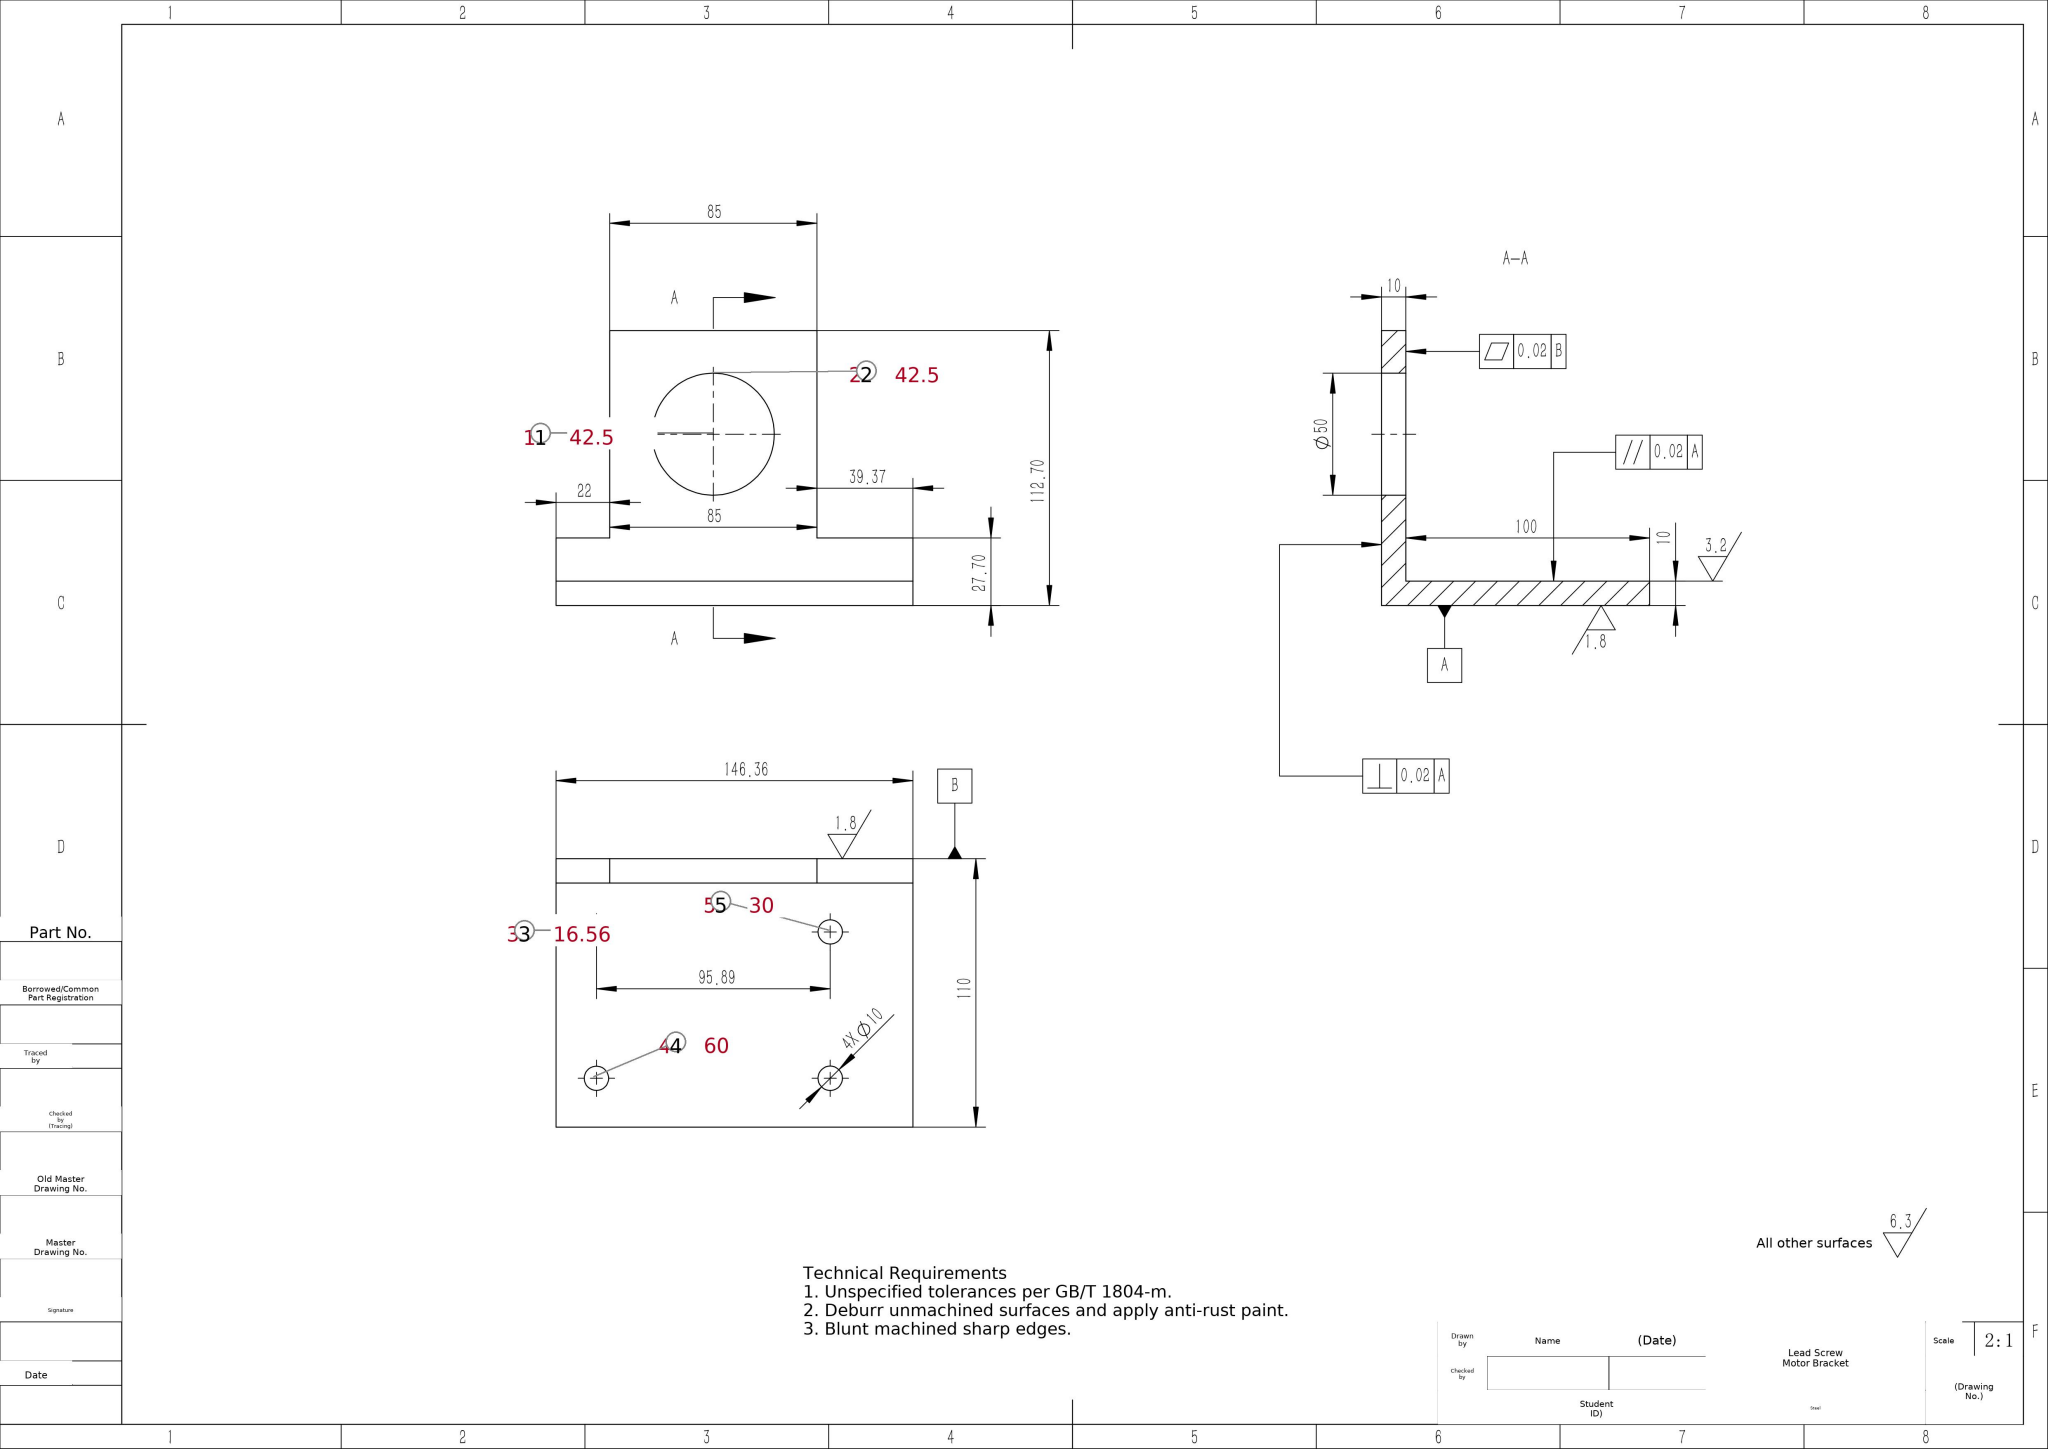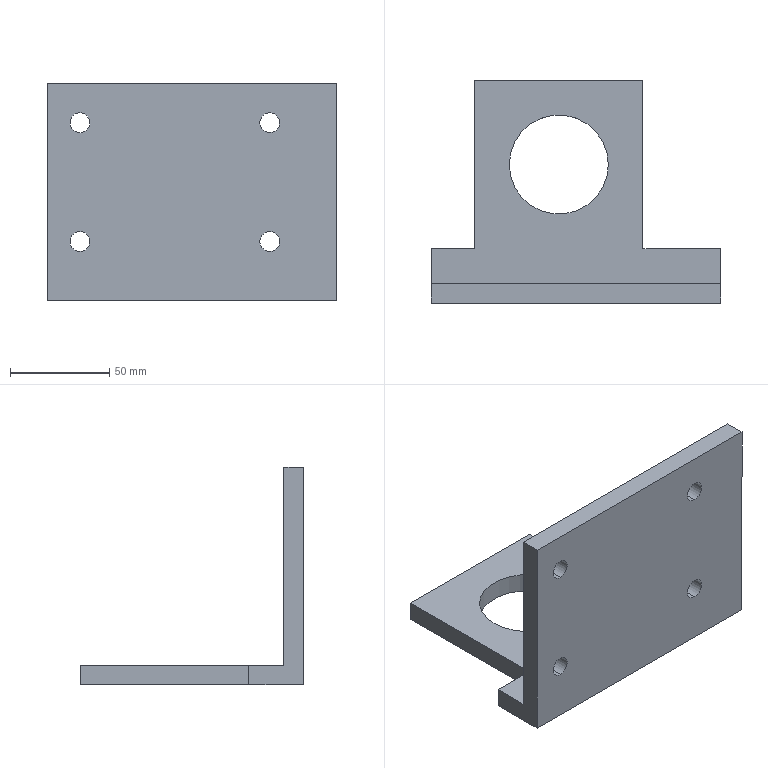Part | SolidWorks | mm | material Steel | 1 solid | 22 faces | box 146.36 x 112.7 x 110 mm | volume 236379 mm3 | plane 12 | cylinder 10 | commonest cylinder face diameters 10 x8 50 x2
STEP:
#1=CARTESIAN_POINT('',(-47.944,-70.2,85.));
#2=VERTEX_POINT('',#1);
#3=CARTESIAN_POINT('',(-47.944,-70.2,95.));
#4=VERTEX_POINT('',#3);
#5=CARTESIAN_POINT('',(-47.944,-70.2,90.));
#6=DIRECTION('',(0.,1.,0.));
#7=DIRECTION('',(0.,0.,1.));
#8=AXIS2_PLACEMENT_3D('',#5,#6,#7);
#9=CIRCLE('',#8,5.);
#10=EDGE_CURVE('',#2,#4,#9,.T.);
#11=ORIENTED_EDGE('',*,*,#10,.F.);
#12=CARTESIAN_POINT('',(-47.944,-60.2,85.));
#13=VERTEX_POINT('',#12);
#14=CARTESIAN_POINT('',(-47.944,-70.2,85.));
#15=DIRECTION('',(0.,1.,0.));
#16=VECTOR('',#15,1000.);
#17=LINE('',#14,#16);
#18=EDGE_CURVE('',#2,#13,#17,.T.);
#19=ORIENTED_EDGE('',*,*,#18,.T.);
#20=CARTESIAN_POINT('',(-47.944,-60.2,95.));
#21=VERTEX_POINT('',#20);
#22=CARTESIAN_POINT('',(-47.944,-60.2,90.));
#23=DIRECTION('',(0.,1.,0.));
#24=DIRECTION('',(0.,0.,1.));
#25=AXIS2_PLACEMENT_3D('',#22,#23,#24);
#26=CIRCLE('',#25,5.);
#27=EDGE_CURVE('',#13,#21,#26,.T.);
#28=ORIENTED_EDGE('',*,*,#27,.T.);
#29=CARTESIAN_POINT('',(-47.944,-70.2,95.));
#30=DIRECTION('',(0.,1.,0.));
#31=VECTOR('',#30,1000.);
#32=LINE('',#29,#31);
#33=EDGE_CURVE('',#4,#21,#32,.T.);
#34=ORIENTED_EDGE('',*,*,#33,.F.);
#35=EDGE_LOOP('',(#11,#19,#28,#34));
#36=FACE_OUTER_BOUND('',#35,.T.);
#37=CARTESIAN_POINT('',(-47.944,-70.2,90.));
#38=DIRECTION('',(0.,1.,0.));
#39=DIRECTION('',(0.,0.,1.));
#40=AXIS2_PLACEMENT_3D('',#37,#38,#39);
#41=CYLINDRICAL_SURFACE('',#40,5.);
#42=ADVANCED_FACE('',(#36),#41,.F.);
#43=CARTESIAN_POINT('',(47.944,-70.2,85.));
#44=VERTEX_POINT('',#43);
#45=CARTESIAN_POINT('',(47.944,-70.2,95.));
#46=VERTEX_POINT('',#45);
#47=CARTESIAN_POINT('',(47.944,-70.2,90.));
#48=DIRECTION('',(0.,1.,0.));
#49=DIRECTION('',(0.,0.,-1.));
#50=AXIS2_PLACEMENT_3D('',#47,#48,#49);
#51=CIRCLE('',#50,5.);
#52=EDGE_CURVE('',#44,#46,#51,.T.);
#53=ORIENTED_EDGE('',*,*,#52,.F.);
#54=CARTESIAN_POINT('',(47.944,-60.2,85.));
#55=VERTEX_POINT('',#54);
#56=CARTESIAN_POINT('',(47.944,-70.2,85.));
#57=DIRECTION('',(0.,1.,0.));
#58=VECTOR('',#57,1000.);
#59=LINE('',#56,#58);
#60=EDGE_CURVE('',#44,#55,#59,.T.);
#61=ORIENTED_EDGE('',*,*,#60,.T.);
#62=CARTESIAN_POINT('',(47.944,-60.2,95.));
#63=VERTEX_POINT('',#62);
#64=CARTESIAN_POINT('',(47.944,-60.2,90.));
#65=DIRECTION('',(0.,1.,0.));
#66=DIRECTION('',(0.,0.,-1.));
#67=AXIS2_PLACEMENT_3D('',#64,#65,#66);
#68=CIRCLE('',#67,5.);
#69=EDGE_CURVE('',#55,#63,#68,.T.);
#70=ORIENTED_EDGE('',*,*,#69,.T.);
#71=CARTESIAN_POINT('',(47.944,-70.2,95.));
#72=DIRECTION('',(0.,1.,0.));
#73=VECTOR('',#72,1000.);
#74=LINE('',#71,#73);
#75=EDGE_CURVE('',#46,#63,#74,.T.);
#76=ORIENTED_EDGE('',*,*,#75,.F.);
#77=EDGE_LOOP('',(#53,#61,#70,#76));
#78=FACE_OUTER_BOUND('',#77,.T.);
#79=CARTESIAN_POINT('',(47.944,-70.2,90.));
#80=DIRECTION('',(0.,1.,0.));
#81=DIRECTION('',(0.,0.,1.));
#82=AXIS2_PLACEMENT_3D('',#79,#80,#81);
#83=CYLINDRICAL_SURFACE('',#82,5.);
#84=ADVANCED_FACE('',(#78),#83,.F.);
#85=CARTESIAN_POINT('',(47.944,-70.2,25.));
#86=VERTEX_POINT('',#85);
#87=CARTESIAN_POINT('',(47.944,-70.2,35.));
#88=VERTEX_POINT('',#87);
#89=CARTESIAN_POINT('',(47.944,-70.2,30.));
#90=DIRECTION('',(0.,1.,0.));
#91=DIRECTION('',(0.,0.,-1.));
#92=AXIS2_PLACEMENT_3D('',#89,#90,#91);
#93=CIRCLE('',#92,5.);
#94=EDGE_CURVE('',#86,#88,#93,.T.);
#95=ORIENTED_EDGE('',*,*,#94,.F.);
#96=CARTESIAN_POINT('',(47.944,-60.2,25.));
#97=VERTEX_POINT('',#96);
#98=CARTESIAN_POINT('',(47.944,-70.2,25.));
#99=DIRECTION('',(0.,1.,0.));
#100=VECTOR('',#99,1000.);
#101=LINE('',#98,#100);
#102=EDGE_CURVE('',#86,#97,#101,.T.);
#103=ORIENTED_EDGE('',*,*,#102,.T.);
#104=CARTESIAN_POINT('',(47.944,-60.2,35.));
#105=VERTEX_POINT('',#104);
#106=CARTESIAN_POINT('',(47.944,-60.2,30.));
#107=DIRECTION('',(0.,1.,0.));
#108=DIRECTION('',(0.,0.,-1.));
#109=AXIS2_PLACEMENT_3D('',#106,#107,#108);
#110=CIRCLE('',#109,5.);
#111=EDGE_CURVE('',#97,#105,#110,.T.);
#112=ORIENTED_EDGE('',*,*,#111,.T.);
#113=CARTESIAN_POINT('',(47.944,-70.2,35.));
#114=DIRECTION('',(0.,1.,0.));
#115=VECTOR('',#114,1000.);
#116=LINE('',#113,#115);
#117=EDGE_CURVE('',#88,#105,#116,.T.);
#118=ORIENTED_EDGE('',*,*,#117,.F.);
#119=EDGE_LOOP('',(#95,#103,#112,#118));
#120=FACE_OUTER_BOUND('',#119,.T.);
#121=CARTESIAN_POINT('',(47.944,-70.2,30.));
#122=DIRECTION('',(0.,1.,0.));
#123=DIRECTION('',(0.,0.,1.));
#124=AXIS2_PLACEMENT_3D('',#121,#122,#123);
#125=CYLINDRICAL_SURFACE('',#124,5.);
#126=ADVANCED_FACE('',(#120),#125,.F.);
#127=CARTESIAN_POINT('',(-47.944,-70.2,25.));
#128=VERTEX_POINT('',#127);
#129=CARTESIAN_POINT('',(-47.944,-70.2,35.));
#130=VERTEX_POINT('',#129);
#131=CARTESIAN_POINT('',(-47.944,-70.2,30.));
#132=DIRECTION('',(0.,1.,0.));
#133=DIRECTION('',(0.,0.,1.));
#134=AXIS2_PLACEMENT_3D('',#131,#132,#133);
#135=CIRCLE('',#134,5.);
#136=EDGE_CURVE('',#128,#130,#135,.T.);
#137=ORIENTED_EDGE('',*,*,#136,.F.);
#138=CARTESIAN_POINT('',(-47.944,-60.2,25.));
#139=VERTEX_POINT('',#138);
#140=CARTESIAN_POINT('',(-47.944,-70.2,25.));
#141=DIRECTION('',(0.,1.,0.));
#142=VECTOR('',#141,1000.);
#143=LINE('',#140,#142);
#144=EDGE_CURVE('',#128,#139,#143,.T.);
#145=ORIENTED_EDGE('',*,*,#144,.T.);
#146=CARTESIAN_POINT('',(-47.944,-60.2,35.));
#147=VERTEX_POINT('',#146);
#148=CARTESIAN_POINT('',(-47.944,-60.2,30.));
#149=DIRECTION('',(0.,1.,0.));
#150=DIRECTION('',(0.,0.,1.));
#151=AXIS2_PLACEMENT_3D('',#148,#149,#150);
#152=CIRCLE('',#151,5.);
#153=EDGE_CURVE('',#139,#147,#152,.T.);
#154=ORIENTED_EDGE('',*,*,#153,.T.);
#155=CARTESIAN_POINT('',(-47.944,-70.2,35.));
#156=DIRECTION('',(0.,1.,0.));
#157=VECTOR('',#156,1000.);
#158=LINE('',#155,#157);
#159=EDGE_CURVE('',#130,#147,#158,.T.);
#160=ORIENTED_EDGE('',*,*,#159,.F.);
#161=EDGE_LOOP('',(#137,#145,#154,#160));
#162=FACE_OUTER_BOUND('',#161,.T.);
#163=CARTESIAN_POINT('',(-47.944,-70.2,30.));
#164=DIRECTION('',(0.,1.,0.));
#165=DIRECTION('',(0.,0.,1.));
#166=AXIS2_PLACEMENT_3D('',#163,#164,#165);
#167=CYLINDRICAL_SURFACE('',#166,5.);
#168=ADVANCED_FACE('',(#162),#167,.F.);
#169=CARTESIAN_POINT('',(-25.,0.,10.));
#170=VERTEX_POINT('',#169);
#171=CARTESIAN_POINT('',(25.,0.,10.));
#172=VERTEX_POINT('',#171);
#173=CARTESIAN_POINT('',(0.,0.,10.));
#174=DIRECTION('',(0.,0.,1.));
#175=DIRECTION('',(1.,0.,0.));
#176=AXIS2_PLACEMENT_3D('',#173,#174,#175);
#177=CIRCLE('',#176,25.);
#178=EDGE_CURVE('',#170,#172,#177,.T.);
#179=ORIENTED_EDGE('',*,*,#178,.T.);
#180=CARTESIAN_POINT('',(25.,0.,0.));
#181=VERTEX_POINT('',#180);
#182=CARTESIAN_POINT('',(25.,0.,10.));
#183=DIRECTION('',(0.,0.,-1.));
#184=VECTOR('',#183,1000.);
#185=LINE('',#182,#184);
#186=EDGE_CURVE('',#172,#181,#185,.T.);
#187=ORIENTED_EDGE('',*,*,#186,.T.);
#188=CARTESIAN_POINT('',(-25.,0.,0.));
#189=VERTEX_POINT('',#188);
#190=CARTESIAN_POINT('',(0.,0.,0.));
#191=DIRECTION('',(0.,0.,1.));
#192=DIRECTION('',(1.,0.,0.));
#193=AXIS2_PLACEMENT_3D('',#190,#191,#192);
#194=CIRCLE('',#193,25.);
#195=EDGE_CURVE('',#189,#181,#194,.T.);
#196=ORIENTED_EDGE('',*,*,#195,.F.);
#197=CARTESIAN_POINT('',(-25.,0.,10.));
#198=DIRECTION('',(0.,0.,-1.));
#199=VECTOR('',#198,1000.);
#200=LINE('',#197,#199);
#201=EDGE_CURVE('',#170,#189,#200,.T.);
#202=ORIENTED_EDGE('',*,*,#201,.F.);
#203=EDGE_LOOP('',(#179,#187,#196,#202));
#204=FACE_OUTER_BOUND('',#203,.T.);
#205=CARTESIAN_POINT('',(0.,0.,10.));
#206=DIRECTION('',(0.,0.,-1.));
#207=DIRECTION('',(-1.,0.,0.));
#208=AXIS2_PLACEMENT_3D('',#205,#206,#207);
#209=CYLINDRICAL_SURFACE('',#208,25.);
#210=ADVANCED_FACE('',(#204),#209,.F.);
#211=ORIENTED_EDGE('',*,*,#178,.F.);
#212=CARTESIAN_POINT('',(0.,0.,10.));
#213=DIRECTION('',(0.,0.,1.));
#214=DIRECTION('',(1.,0.,0.));
#215=AXIS2_PLACEMENT_3D('',#212,#213,#214);
#216=CIRCLE('',#215,25.);
#217=EDGE_CURVE('',#172,#170,#216,.T.);
#218=ORIENTED_EDGE('',*,*,#217,.F.);
#219=EDGE_LOOP('',(#211,#218));
#220=FACE_BOUND('',#219,.T.);
#221=CARTESIAN_POINT('',(-42.5,-42.5,10.));
#222=VERTEX_POINT('',#221);
#223=CARTESIAN_POINT('',(-64.496,-42.5,10.));
#224=VERTEX_POINT('',#223);
#225=CARTESIAN_POINT('',(-42.5,-42.5,10.));
#226=DIRECTION('',(-1.,0.,0.));
#227=VECTOR('',#226,1000.);
#228=LINE('',#225,#227);
#229=EDGE_CURVE('',#222,#224,#228,.T.);
#230=ORIENTED_EDGE('',*,*,#229,.T.);
#231=CARTESIAN_POINT('',(-64.496,-60.2,10.));
#232=VERTEX_POINT('',#231);
#233=CARTESIAN_POINT('',(-64.496,-60.2,10.));
#234=DIRECTION('',(0.,1.,0.));
#235=VECTOR('',#234,1000.);
#236=LINE('',#233,#235);
#237=EDGE_CURVE('',#232,#224,#236,.T.);
#238=ORIENTED_EDGE('',*,*,#237,.F.);
#239=CARTESIAN_POINT('',(81.866,-60.2,10.));
#240=VERTEX_POINT('',#239);
#241=CARTESIAN_POINT('',(-81.866,-60.2,10.));
#242=DIRECTION('',(-1.,0.,0.));
#243=VECTOR('',#242,1000.);
#244=LINE('',#241,#243);
#245=EDGE_CURVE('',#240,#232,#244,.T.);
#246=ORIENTED_EDGE('',*,*,#245,.F.);
#247=CARTESIAN_POINT('',(81.866,-42.5,10.));
#248=VERTEX_POINT('',#247);
#249=CARTESIAN_POINT('',(81.866,-42.5,10.));
#250=DIRECTION('',(-0.,1.,0.));
#251=VECTOR('',#250,1000.);
#252=LINE('',#249,#251);
#253=EDGE_CURVE('',#240,#248,#252,.T.);
#254=ORIENTED_EDGE('',*,*,#253,.T.);
#255=CARTESIAN_POINT('',(42.5,-42.5,10.));
#256=VERTEX_POINT('',#255);
#257=CARTESIAN_POINT('',(42.5,-42.5,10.));
#258=DIRECTION('',(-1.,-0.,0.));
#259=VECTOR('',#258,1000.);
#260=LINE('',#257,#259);
#261=EDGE_CURVE('',#248,#256,#260,.T.);
#262=ORIENTED_EDGE('',*,*,#261,.T.);
#263=CARTESIAN_POINT('',(42.5,42.5,10.));
#264=VERTEX_POINT('',#263);
#265=CARTESIAN_POINT('',(42.5,42.5,10.));
#266=DIRECTION('',(-0.,1.,0.));
#267=VECTOR('',#266,1000.);
#268=LINE('',#265,#267);
#269=EDGE_CURVE('',#256,#264,#268,.T.);
#270=ORIENTED_EDGE('',*,*,#269,.T.);
#271=CARTESIAN_POINT('',(-42.5,42.5,10.));
#272=VERTEX_POINT('',#271);
#273=CARTESIAN_POINT('',(42.5,42.5,10.));
#274=DIRECTION('',(-1.,-0.,0.));
#275=VECTOR('',#274,1000.);
#276=LINE('',#273,#275);
#277=EDGE_CURVE('',#264,#272,#276,.T.);
#278=ORIENTED_EDGE('',*,*,#277,.T.);
#279=CARTESIAN_POINT('',(-42.5,42.5,10.));
#280=DIRECTION('',(0.,-1.,0.));
#281=VECTOR('',#280,1000.);
#282=LINE('',#279,#281);
#283=EDGE_CURVE('',#272,#222,#282,.T.);
#284=ORIENTED_EDGE('',*,*,#283,.T.);
#285=EDGE_LOOP('',(#230,#238,#246,#254,#262,#270,#278,#284));
#286=FACE_OUTER_BOUND('',#285,.T.);
#287=CARTESIAN_POINT('',(0.,0.,10.));
#288=DIRECTION('',(0.,0.,1.));
#289=DIRECTION('',(1.,0.,0.));
#290=AXIS2_PLACEMENT_3D('',#287,#288,#289);
#291=PLANE('',#290);
#292=ADVANCED_FACE('',(#220,#286),#291,.T.);
#293=ORIENTED_EDGE('',*,*,#195,.T.);
#294=CARTESIAN_POINT('',(0.,0.,0.));
#295=DIRECTION('',(0.,0.,1.));
#296=DIRECTION('',(1.,0.,0.));
#297=AXIS2_PLACEMENT_3D('',#294,#295,#296);
#298=CIRCLE('',#297,25.);
#299=EDGE_CURVE('',#181,#189,#298,.T.);
#300=ORIENTED_EDGE('',*,*,#299,.T.);
#301=EDGE_LOOP('',(#293,#300));
#302=FACE_BOUND('',#301,.T.);
#303=CARTESIAN_POINT('',(-64.496,-42.5,0.));
#304=VERTEX_POINT('',#303);
#305=CARTESIAN_POINT('',(-64.496,-70.2,0.));
#306=VERTEX_POINT('',#305);
#307=CARTESIAN_POINT('',(-64.496,-42.5,0.));
#308=DIRECTION('',(0.,-1.,0.));
#309=VECTOR('',#308,1000.);
#310=LINE('',#307,#309);
#311=EDGE_CURVE('',#304,#306,#310,.T.);
#312=ORIENTED_EDGE('',*,*,#311,.F.);
#313=CARTESIAN_POINT('',(-42.5,-42.5,0.));
#314=VERTEX_POINT('',#313);
#315=CARTESIAN_POINT('',(-42.5,-42.5,0.));
#316=DIRECTION('',(-1.,0.,0.));
#317=VECTOR('',#316,1000.);
#318=LINE('',#315,#317);
#319=EDGE_CURVE('',#314,#304,#318,.T.);
#320=ORIENTED_EDGE('',*,*,#319,.F.);
#321=CARTESIAN_POINT('',(-42.5,42.5,0.));
#322=VERTEX_POINT('',#321);
#323=CARTESIAN_POINT('',(-42.5,42.5,0.));
#324=DIRECTION('',(0.,-1.,0.));
#325=VECTOR('',#324,1000.);
#326=LINE('',#323,#325);
#327=EDGE_CURVE('',#322,#314,#326,.T.);
#328=ORIENTED_EDGE('',*,*,#327,.F.);
#329=CARTESIAN_POINT('',(42.5,42.5,0.));
#330=VERTEX_POINT('',#329);
#331=CARTESIAN_POINT('',(42.5,42.5,0.));
#332=DIRECTION('',(-1.,-0.,0.));
#333=VECTOR('',#332,1000.);
#334=LINE('',#331,#333);
#335=EDGE_CURVE('',#330,#322,#334,.T.);
#336=ORIENTED_EDGE('',*,*,#335,.F.);
#337=CARTESIAN_POINT('',(42.5,-42.5,0.));
#338=VERTEX_POINT('',#337);
#339=CARTESIAN_POINT('',(42.5,42.5,0.));
#340=DIRECTION('',(-0.,1.,0.));
#341=VECTOR('',#340,1000.);
#342=LINE('',#339,#341);
#343=EDGE_CURVE('',#338,#330,#342,.T.);
#344=ORIENTED_EDGE('',*,*,#343,.F.);
#345=CARTESIAN_POINT('',(81.866,-42.5,0.));
#346=VERTEX_POINT('',#345);
#347=CARTESIAN_POINT('',(42.5,-42.5,0.));
#348=DIRECTION('',(-1.,-0.,0.));
#349=VECTOR('',#348,1000.);
#350=LINE('',#347,#349);
#351=EDGE_CURVE('',#346,#338,#350,.T.);
#352=ORIENTED_EDGE('',*,*,#351,.F.);
#353=CARTESIAN_POINT('',(81.866,-70.2,0.));
#354=VERTEX_POINT('',#353);
#355=CARTESIAN_POINT('',(81.866,-42.5,0.));
#356=DIRECTION('',(-0.,1.,0.));
#357=VECTOR('',#356,1000.);
#358=LINE('',#355,#357);
#359=EDGE_CURVE('',#354,#346,#358,.T.);
#360=ORIENTED_EDGE('',*,*,#359,.F.);
#361=CARTESIAN_POINT('',(-81.866,-70.2,0.));
#362=DIRECTION('',(1.,0.,0.));
#363=VECTOR('',#362,1000.);
#364=LINE('',#361,#363);
#365=EDGE_CURVE('',#306,#354,#364,.T.);
#366=ORIENTED_EDGE('',*,*,#365,.F.);
#367=EDGE_LOOP('',(#312,#320,#328,#336,#344,#352,#360,#366));
#368=FACE_OUTER_BOUND('',#367,.T.);
#369=CARTESIAN_POINT('',(0.,0.,0.));
#370=DIRECTION('',(0.,0.,1.));
#371=DIRECTION('',(1.,0.,0.));
#372=AXIS2_PLACEMENT_3D('',#369,#370,#371);
#373=PLANE('',#372);
#374=ADVANCED_FACE('',(#302,#368),#373,.F.);
#375=CARTESIAN_POINT('',(-64.496,-42.5,10.));
#376=DIRECTION('',(0.,0.,-1.));
#377=VECTOR('',#376,1000.);
#378=LINE('',#375,#377);
#379=EDGE_CURVE('',#224,#304,#378,.T.);
#380=ORIENTED_EDGE('',*,*,#379,.F.);
#381=ORIENTED_EDGE('',*,*,#229,.F.);
#382=CARTESIAN_POINT('',(-42.5,-42.5,10.));
#383=DIRECTION('',(0.,0.,-1.));
#384=VECTOR('',#383,1000.);
#385=LINE('',#382,#384);
#386=EDGE_CURVE('',#222,#314,#385,.T.);
#387=ORIENTED_EDGE('',*,*,#386,.T.);
#388=ORIENTED_EDGE('',*,*,#319,.T.);
#389=EDGE_LOOP('',(#380,#381,#387,#388));
#390=FACE_OUTER_BOUND('',#389,.T.);
#391=CARTESIAN_POINT('',(-42.5,-42.5,10.));
#392=DIRECTION('',(0.,-1.,0.));
#393=DIRECTION('',(0.,0.,-1.));
#394=AXIS2_PLACEMENT_3D('',#391,#392,#393);
#395=PLANE('',#394);
#396=ADVANCED_FACE('',(#390),#395,.F.);
#397=CARTESIAN_POINT('',(-47.944,-70.2,90.));
#398=DIRECTION('',(0.,1.,0.));
#399=DIRECTION('',(0.,0.,1.));
#400=AXIS2_PLACEMENT_3D('',#397,#398,#399);
#401=CIRCLE('',#400,5.);
#402=EDGE_CURVE('',#4,#2,#401,.T.);
#403=ORIENTED_EDGE('',*,*,#402,.T.);
#404=ORIENTED_EDGE('',*,*,#10,.T.);
#405=EDGE_LOOP('',(#403,#404));
#406=FACE_BOUND('',#405,.T.);
#407=CARTESIAN_POINT('',(47.944,-70.2,90.));
#408=DIRECTION('',(0.,1.,0.));
#409=DIRECTION('',(0.,0.,-1.));
#410=AXIS2_PLACEMENT_3D('',#407,#408,#409);
#411=CIRCLE('',#410,5.);
#412=EDGE_CURVE('',#46,#44,#411,.T.);
#413=ORIENTED_EDGE('',*,*,#412,.T.);
#414=ORIENTED_EDGE('',*,*,#52,.T.);
#415=EDGE_LOOP('',(#413,#414));
#416=FACE_BOUND('',#415,.T.);
#417=CARTESIAN_POINT('',(47.944,-70.2,30.));
#418=DIRECTION('',(0.,1.,0.));
#419=DIRECTION('',(0.,0.,-1.));
#420=AXIS2_PLACEMENT_3D('',#417,#418,#419);
#421=CIRCLE('',#420,5.);
#422=EDGE_CURVE('',#88,#86,#421,.T.);
#423=ORIENTED_EDGE('',*,*,#422,.T.);
#424=ORIENTED_EDGE('',*,*,#94,.T.);
#425=EDGE_LOOP('',(#423,#424));
#426=FACE_BOUND('',#425,.T.);
#427=CARTESIAN_POINT('',(-47.944,-70.2,30.));
#428=DIRECTION('',(0.,1.,0.));
#429=DIRECTION('',(0.,0.,1.));
#430=AXIS2_PLACEMENT_3D('',#427,#428,#429);
#431=CIRCLE('',#430,5.);
#432=EDGE_CURVE('',#130,#128,#431,.T.);
#433=ORIENTED_EDGE('',*,*,#432,.T.);
#434=ORIENTED_EDGE('',*,*,#136,.T.);
#435=EDGE_LOOP('',(#433,#434));
#436=FACE_BOUND('',#435,.T.);
#437=CARTESIAN_POINT('',(-64.496,-70.2,110.));
#438=VERTEX_POINT('',#437);
#439=CARTESIAN_POINT('',(-64.496,-70.2,0.));
#440=DIRECTION('',(0.,0.,1.));
#441=VECTOR('',#440,1000.);
#442=LINE('',#439,#441);
#443=EDGE_CURVE('',#306,#438,#442,.T.);
#444=ORIENTED_EDGE('',*,*,#443,.F.);
#445=ORIENTED_EDGE('',*,*,#365,.T.);
#446=CARTESIAN_POINT('',(81.866,-70.2,110.));
#447=VERTEX_POINT('',#446);
#448=CARTESIAN_POINT('',(81.866,-70.2,10.));
#449=DIRECTION('',(0.,0.,-1.));
#450=VECTOR('',#449,1000.);
#451=LINE('',#448,#450);
#452=EDGE_CURVE('',#447,#354,#451,.T.);
#453=ORIENTED_EDGE('',*,*,#452,.F.);
#454=CARTESIAN_POINT('',(-81.866,-70.2,110.));
#455=DIRECTION('',(1.,0.,0.));
#456=VECTOR('',#455,1000.);
#457=LINE('',#454,#456);
#458=EDGE_CURVE('',#438,#447,#457,.T.);
#459=ORIENTED_EDGE('',*,*,#458,.F.);
#460=EDGE_LOOP('',(#444,#445,#453,#459));
#461=FACE_OUTER_BOUND('',#460,.T.);
#462=CARTESIAN_POINT('',(-81.866,-70.2,10.));
#463=DIRECTION('',(-0.,1.,0.));
#464=DIRECTION('',(-1.,-0.,0.));
#465=AXIS2_PLACEMENT_3D('',#462,#463,#464);
#466=PLANE('',#465);
#467=ADVANCED_FACE('',(#406,#416,#426,#436,#461),#466,.F.);
#468=CARTESIAN_POINT('',(-47.944,-60.2,90.));
#469=DIRECTION('',(0.,1.,0.));
#470=DIRECTION('',(0.,0.,1.));
#471=AXIS2_PLACEMENT_3D('',#468,#469,#470);
#472=CIRCLE('',#471,5.);
#473=EDGE_CURVE('',#21,#13,#472,.T.);
#474=ORIENTED_EDGE('',*,*,#473,.F.);
#475=ORIENTED_EDGE('',*,*,#27,.F.);
#476=EDGE_LOOP('',(#474,#475));
#477=FACE_BOUND('',#476,.T.);
#478=CARTESIAN_POINT('',(47.944,-60.2,90.));
#479=DIRECTION('',(0.,1.,0.));
#480=DIRECTION('',(0.,0.,-1.));
#481=AXIS2_PLACEMENT_3D('',#478,#479,#480);
#482=CIRCLE('',#481,5.);
#483=EDGE_CURVE('',#63,#55,#482,.T.);
#484=ORIENTED_EDGE('',*,*,#483,.F.);
#485=ORIENTED_EDGE('',*,*,#69,.F.);
#486=EDGE_LOOP('',(#484,#485));
#487=FACE_BOUND('',#486,.T.);
#488=CARTESIAN_POINT('',(47.944,-60.2,30.));
#489=DIRECTION('',(0.,1.,0.));
#490=DIRECTION('',(0.,0.,-1.));
#491=AXIS2_PLACEMENT_3D('',#488,#489,#490);
#492=CIRCLE('',#491,5.);
#493=EDGE_CURVE('',#105,#97,#492,.T.);
#494=ORIENTED_EDGE('',*,*,#493,.F.);
#495=ORIENTED_EDGE('',*,*,#111,.F.);
#496=EDGE_LOOP('',(#494,#495));
#497=FACE_BOUND('',#496,.T.);
#498=CARTESIAN_POINT('',(-47.944,-60.2,30.));
#499=DIRECTION('',(0.,1.,0.));
#500=DIRECTION('',(0.,0.,1.));
#501=AXIS2_PLACEMENT_3D('',#498,#499,#500);
#502=CIRCLE('',#501,5.);
#503=EDGE_CURVE('',#147,#139,#502,.T.);
#504=ORIENTED_EDGE('',*,*,#503,.F.);
#505=ORIENTED_EDGE('',*,*,#153,.F.);
#506=EDGE_LOOP('',(#504,#505));
#507=FACE_BOUND('',#506,.T.);
#508=CARTESIAN_POINT('',(-64.496,-60.2,110.));
#509=VERTEX_POINT('',#508);
#510=CARTESIAN_POINT('',(-64.496,-60.2,110.));
#511=DIRECTION('',(0.,0.,-1.));
#512=VECTOR('',#511,1000.);
#513=LINE('',#510,#512);
#514=EDGE_CURVE('',#509,#232,#513,.T.);
#515=ORIENTED_EDGE('',*,*,#514,.F.);
#516=CARTESIAN_POINT('',(81.866,-60.2,110.));
#517=VERTEX_POINT('',#516);
#518=CARTESIAN_POINT('',(-81.866,-60.2,110.));
#519=DIRECTION('',(-1.,0.,0.));
#520=VECTOR('',#519,1000.);
#521=LINE('',#518,#520);
#522=EDGE_CURVE('',#517,#509,#521,.T.);
#523=ORIENTED_EDGE('',*,*,#522,.F.);
#524=CARTESIAN_POINT('',(81.866,-60.2,110.));
#525=DIRECTION('',(0.,0.,-1.));
#526=VECTOR('',#525,1000.);
#527=LINE('',#524,#526);
#528=EDGE_CURVE('',#517,#240,#527,.T.);
#529=ORIENTED_EDGE('',*,*,#528,.T.);
#530=ORIENTED_EDGE('',*,*,#245,.T.);
#531=EDGE_LOOP('',(#515,#523,#529,#530));
#532=FACE_OUTER_BOUND('',#531,.T.);
#533=CARTESIAN_POINT('',(-81.866,-60.2,110.));
#534=DIRECTION('',(0.,-1.,0.));
#535=DIRECTION('',(0.,0.,-1.));
#536=AXIS2_PLACEMENT_3D('',#533,#534,#535);
#537=PLANE('',#536);
#538=ADVANCED_FACE('',(#477,#487,#497,#507,#532),#537,.F.);
#539=CARTESIAN_POINT('',(-64.496,-70.2,110.));
#540=DIRECTION('',(0.,1.,0.));
#541=VECTOR('',#540,1000.);
#542=LINE('',#539,#541);
#543=EDGE_CURVE('',#438,#509,#542,.T.);
#544=ORIENTED_EDGE('',*,*,#543,.F.);
#545=ORIENTED_EDGE('',*,*,#458,.T.);
#546=CARTESIAN_POINT('',(81.866,-70.2,110.));
#547=DIRECTION('',(0.,1.,0.));
#548=VECTOR('',#547,1000.);
#549=LINE('',#546,#548);
#550=EDGE_CURVE('',#447,#517,#549,.T.);
#551=ORIENTED_EDGE('',*,*,#550,.T.);
#552=ORIENTED_EDGE('',*,*,#522,.T.);
#553=EDGE_LOOP('',(#544,#545,#551,#552));
#554=FACE_OUTER_BOUND('',#553,.T.);
#555=CARTESIAN_POINT('',(0.,0.,110.));
#556=DIRECTION('',(0.,0.,-1.));
#557=DIRECTION('',(-1.,0.,0.));
#558=AXIS2_PLACEMENT_3D('',#555,#556,#557);
#559=PLANE('',#558);
#560=ADVANCED_FACE('',(#554),#559,.F.);
#561=ORIENTED_EDGE('',*,*,#359,.T.);
#562=CARTESIAN_POINT('',(81.866,-42.5,10.));
#563=DIRECTION('',(0.,0.,-1.));
#564=VECTOR('',#563,1000.);
#565=LINE('',#562,#564);
#566=EDGE_CURVE('',#248,#346,#565,.T.);
#567=ORIENTED_EDGE('',*,*,#566,.F.);
#568=ORIENTED_EDGE('',*,*,#253,.F.);
#569=ORIENTED_EDGE('',*,*,#528,.F.);
#570=ORIENTED_EDGE('',*,*,#550,.F.);
#571=ORIENTED_EDGE('',*,*,#452,.T.);
#572=EDGE_LOOP('',(#561,#567,#568,#569,#570,#571));
#573=FACE_OUTER_BOUND('',#572,.T.);
#574=CARTESIAN_POINT('',(81.866,-42.5,10.));
#575=DIRECTION('',(-1.,-0.,0.));
#576=DIRECTION('',(0.,-1.,0.));
#577=AXIS2_PLACEMENT_3D('',#574,#575,#576);
#578=PLANE('',#577);
#579=ADVANCED_FACE('',(#573),#578,.F.);
#580=ORIENTED_EDGE('',*,*,#351,.T.);
#581=CARTESIAN_POINT('',(42.5,-42.5,10.));
#582=DIRECTION('',(0.,0.,-1.));
#583=VECTOR('',#582,1000.);
#584=LINE('',#581,#583);
#585=EDGE_CURVE('',#256,#338,#584,.T.);
#586=ORIENTED_EDGE('',*,*,#585,.F.);
#587=ORIENTED_EDGE('',*,*,#261,.F.);
#588=ORIENTED_EDGE('',*,*,#566,.T.);
#589=EDGE_LOOP('',(#580,#586,#587,#588));
#590=FACE_OUTER_BOUND('',#589,.T.);
#591=CARTESIAN_POINT('',(42.5,-42.5,10.));
#592=DIRECTION('',(0.,-1.,0.));
#593=DIRECTION('',(1.,0.,0.));
#594=AXIS2_PLACEMENT_3D('',#591,#592,#593);
#595=PLANE('',#594);
#596=ADVANCED_FACE('',(#590),#595,.F.);
#597=ORIENTED_EDGE('',*,*,#343,.T.);
#598=CARTESIAN_POINT('',(42.5,42.5,10.));
#599=DIRECTION('',(0.,0.,-1.));
#600=VECTOR('',#599,1000.);
#601=LINE('',#598,#600);
#602=EDGE_CURVE('',#264,#330,#601,.T.);
#603=ORIENTED_EDGE('',*,*,#602,.F.);
#604=ORIENTED_EDGE('',*,*,#269,.F.);
#605=ORIENTED_EDGE('',*,*,#585,.T.);
#606=EDGE_LOOP('',(#597,#603,#604,#605));
#607=FACE_OUTER_BOUND('',#606,.T.);
#608=CARTESIAN_POINT('',(42.5,42.5,10.));
#609=DIRECTION('',(-1.,-0.,0.));
#610=DIRECTION('',(0.,-1.,0.));
#611=AXIS2_PLACEMENT_3D('',#608,#609,#610);
#612=PLANE('',#611);
#613=ADVANCED_FACE('',(#607),#612,.F.);
#614=ORIENTED_EDGE('',*,*,#335,.T.);
#615=CARTESIAN_POINT('',(-42.5,42.5,10.));
#616=DIRECTION('',(0.,0.,-1.));
#617=VECTOR('',#616,1000.);
#618=LINE('',#615,#617);
#619=EDGE_CURVE('',#272,#322,#618,.T.);
#620=ORIENTED_EDGE('',*,*,#619,.F.);
#621=ORIENTED_EDGE('',*,*,#277,.F.);
#622=ORIENTED_EDGE('',*,*,#602,.T.);
#623=EDGE_LOOP('',(#614,#620,#621,#622));
#624=FACE_OUTER_BOUND('',#623,.T.);
#625=CARTESIAN_POINT('',(42.5,42.5,10.));
#626=DIRECTION('',(0.,-1.,0.));
#627=DIRECTION('',(1.,0.,0.));
#628=AXIS2_PLACEMENT_3D('',#625,#626,#627);
#629=PLANE('',#628);
#630=ADVANCED_FACE('',(#624),#629,.F.);
#631=ORIENTED_EDGE('',*,*,#327,.T.);
#632=ORIENTED_EDGE('',*,*,#386,.F.);
#633=ORIENTED_EDGE('',*,*,#283,.F.);
#634=ORIENTED_EDGE('',*,*,#619,.T.);
#635=EDGE_LOOP('',(#631,#632,#633,#634));
#636=FACE_OUTER_BOUND('',#635,.T.);
#637=CARTESIAN_POINT('',(-42.5,42.5,10.));
#638=DIRECTION('',(1.,0.,0.));
#639=DIRECTION('',(-0.,1.,0.));
#640=AXIS2_PLACEMENT_3D('',#637,#638,#639);
#641=PLANE('',#640);
#642=ADVANCED_FACE('',(#636),#641,.F.);
#643=ORIENTED_EDGE('',*,*,#186,.F.);
#644=ORIENTED_EDGE('',*,*,#217,.T.);
#645=ORIENTED_EDGE('',*,*,#201,.T.);
#646=ORIENTED_EDGE('',*,*,#299,.F.);
#647=EDGE_LOOP('',(#643,#644,#645,#646));
#648=FACE_OUTER_BOUND('',#647,.T.);
#649=CARTESIAN_POINT('',(0.,0.,10.));
#650=DIRECTION('',(0.,0.,-1.));
#651=DIRECTION('',(-1.,0.,0.));
#652=AXIS2_PLACEMENT_3D('',#649,#650,#651);
#653=CYLINDRICAL_SURFACE('',#652,25.);
#654=ADVANCED_FACE('',(#648),#653,.F.);
#655=ORIENTED_EDGE('',*,*,#379,.T.);
#656=ORIENTED_EDGE('',*,*,#311,.T.);
#657=ORIENTED_EDGE('',*,*,#443,.T.);
#658=ORIENTED_EDGE('',*,*,#543,.T.);
#659=ORIENTED_EDGE('',*,*,#514,.T.);
#660=ORIENTED_EDGE('',*,*,#237,.T.);
#661=EDGE_LOOP('',(#655,#656,#657,#658,#659,#660));
#662=FACE_OUTER_BOUND('',#661,.T.);
#663=CARTESIAN_POINT('',(-64.496,0.,0.));
#664=DIRECTION('',(-1.,0.,0.));
#665=DIRECTION('',(0.,0.,1.));
#666=AXIS2_PLACEMENT_3D('',#663,#664,#665);
#667=PLANE('',#666);
#668=ADVANCED_FACE('',(#662),#667,.T.);
#669=ORIENTED_EDGE('',*,*,#144,.F.);
#670=ORIENTED_EDGE('',*,*,#432,.F.);
#671=ORIENTED_EDGE('',*,*,#159,.T.);
#672=ORIENTED_EDGE('',*,*,#503,.T.);
#673=EDGE_LOOP('',(#669,#670,#671,#672));
#674=FACE_OUTER_BOUND('',#673,.T.);
#675=CARTESIAN_POINT('',(-47.944,-70.2,30.));
#676=DIRECTION('',(0.,1.,0.));
#677=DIRECTION('',(0.,0.,1.));
#678=AXIS2_PLACEMENT_3D('',#675,#676,#677);
#679=CYLINDRICAL_SURFACE('',#678,5.);
#680=ADVANCED_FACE('',(#674),#679,.F.);
#681=ORIENTED_EDGE('',*,*,#102,.F.);
#682=ORIENTED_EDGE('',*,*,#422,.F.);
#683=ORIENTED_EDGE('',*,*,#117,.T.);
#684=ORIENTED_EDGE('',*,*,#493,.T.);
#685=EDGE_LOOP('',(#681,#682,#683,#684));
#686=FACE_OUTER_BOUND('',#685,.T.);
#687=CARTESIAN_POINT('',(47.944,-70.2,30.));
#688=DIRECTION('',(0.,1.,0.));
#689=DIRECTION('',(0.,0.,1.));
#690=AXIS2_PLACEMENT_3D('',#687,#688,#689);
#691=CYLINDRICAL_SURFACE('',#690,5.);
#692=ADVANCED_FACE('',(#686),#691,.F.);
#693=ORIENTED_EDGE('',*,*,#60,.F.);
#694=ORIENTED_EDGE('',*,*,#412,.F.);
#695=ORIENTED_EDGE('',*,*,#75,.T.);
#696=ORIENTED_EDGE('',*,*,#483,.T.);
#697=EDGE_LOOP('',(#693,#694,#695,#696));
#698=FACE_OUTER_BOUND('',#697,.T.);
#699=CARTESIAN_POINT('',(47.944,-70.2,90.));
#700=DIRECTION('',(0.,1.,0.));
#701=DIRECTION('',(0.,0.,1.));
#702=AXIS2_PLACEMENT_3D('',#699,#700,#701);
#703=CYLINDRICAL_SURFACE('',#702,5.);
#704=ADVANCED_FACE('',(#698),#703,.F.);
#705=ORIENTED_EDGE('',*,*,#18,.F.);
#706=ORIENTED_EDGE('',*,*,#402,.F.);
#707=ORIENTED_EDGE('',*,*,#33,.T.);
#708=ORIENTED_EDGE('',*,*,#473,.T.);
#709=EDGE_LOOP('',(#705,#706,#707,#708));
#710=FACE_OUTER_BOUND('',#709,.T.);
#711=CARTESIAN_POINT('',(-47.944,-70.2,90.));
#712=DIRECTION('',(0.,1.,0.));
#713=DIRECTION('',(0.,0.,1.));
#714=AXIS2_PLACEMENT_3D('',#711,#712,#713);
#715=CYLINDRICAL_SURFACE('',#714,5.);
#716=ADVANCED_FACE('',(#710),#715,.F.);
#717=CLOSED_SHELL('',(#42,#84,#126,#168,#210,#292,#374,#396,#467,#538,#560,#579,#596,#613,#630,#642,#654,#668,#680,#692,#704,#716));
#718=MANIFOLD_SOLID_BREP('',#717);
#719=CARTESIAN_POINT('',(0.,0.,0.));
#720=DIRECTION('',(0.,0.,1.));
#721=DIRECTION('',(1.,0.,0.));
#722=AXIS2_PLACEMENT_3D('',#719,#720,#721);
#723=(LENGTH_UNIT()NAMED_UNIT(*)SI_UNIT(.MILLI.,.METRE.));
#724=UNCERTAINTY_MEASURE_WITH_UNIT(LENGTH_MEASURE(0.00001),#723,'','');
#725=(NAMED_UNIT(*)PLANE_ANGLE_UNIT()SI_UNIT($,.RADIAN.));
#726=(NAMED_UNIT(*)SI_UNIT($,.STERADIAN.)SOLID_ANGLE_UNIT());
#727=(GEOMETRIC_REPRESENTATION_CONTEXT(3)GLOBAL_UNCERTAINTY_ASSIGNED_CONTEXT((#724))GLOBAL_UNIT_ASSIGNED_CONTEXT((#723,#725,#726))REPRESENTATION_CONTEXT('',''));
#728=ADVANCED_BREP_SHAPE_REPRESENTATION('',(#718,#722),#727);